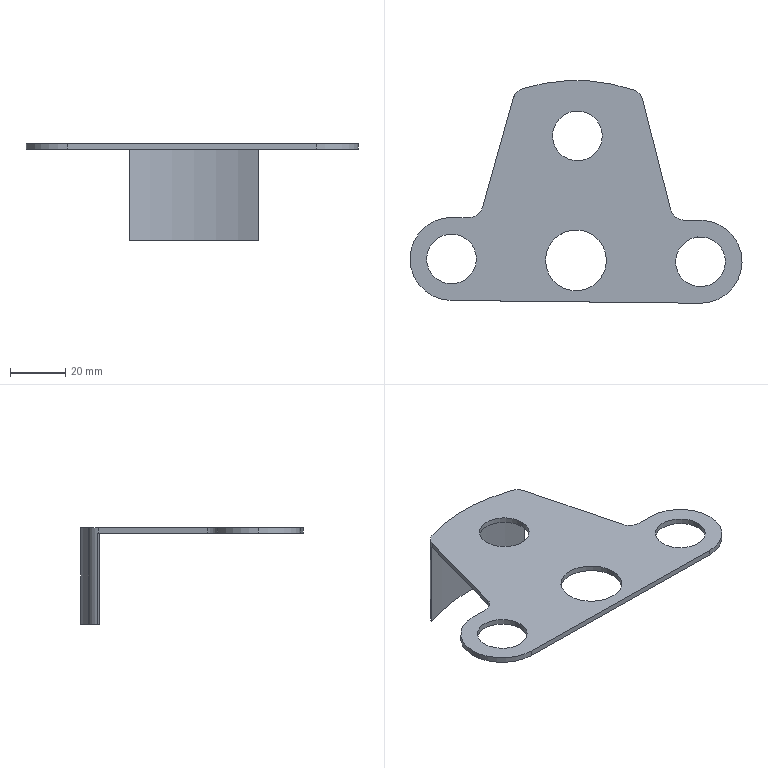Component | SolidWorks | JF21-80.2-34-1-SOLID1-1 | 1 solid | 26 faces | box 119.99 x 80.51 x 35 mm | volume 13117 mm3 | cylinder 18 | plane 8 | commonest cylinder face diameters 18 x6 30 x4 10 x4 22 x2 130 x1 126 x1
STEP:
#1=COLOUR_RGB('',0.7922,0.8196,0.9333);
#2=FILL_AREA_STYLE_COLOUR('',#1);
#3=FILL_AREA_STYLE('',(#2));
#4=SURFACE_STYLE_FILL_AREA(#3);
#5=SURFACE_SIDE_STYLE('',(#4));
#6=SURFACE_STYLE_USAGE(.BOTH.,#5);
#7=PRESENTATION_STYLE_ASSIGNMENT((#6));
#8=CARTESIAN_POINT('',(-1.765,0.6105,-11.063));
#9=VERTEX_POINT('',#8);
#10=CARTESIAN_POINT('',(-2.362,0.02663,-11.063));
#11=VERTEX_POINT('',#10);
#12=CARTESIAN_POINT('',(-1.772,0.01997,-11.063));
#13=DIRECTION('',(0.,0.,1.));
#14=DIRECTION('',(0.9999,-0.01127,0.));
#15=AXIS2_PLACEMENT_3D('',#12,#13,#14);
#16=CIRCLE('',#15,0.5906);
#17=EDGE_CURVE('',#9,#11,#16,.T.);
#18=ORIENTED_EDGE('',*,*,#17,.T.);
#19=CARTESIAN_POINT('',(-2.362,0.02663,-10.984));
#20=VERTEX_POINT('',#19);
#21=CARTESIAN_POINT('',(-2.362,0.02663,-11.063));
#22=DIRECTION('',(0.,0.,1.));
#23=VECTOR('',#22,39.37);
#24=LINE('',#21,#23);
#25=EDGE_CURVE('',#11,#20,#24,.T.);
#26=ORIENTED_EDGE('',*,*,#25,.T.);
#27=CARTESIAN_POINT('',(-1.765,0.6105,-10.984));
#28=VERTEX_POINT('',#27);
#29=CARTESIAN_POINT('',(-1.772,0.01997,-10.984));
#30=DIRECTION('',(0.,0.,1.));
#31=DIRECTION('',(0.9999,-0.01127,0.));
#32=AXIS2_PLACEMENT_3D('',#29,#30,#31);
#33=CIRCLE('',#32,0.5906);
#34=EDGE_CURVE('',#28,#20,#33,.T.);
#35=ORIENTED_EDGE('',*,*,#34,.F.);
#36=CARTESIAN_POINT('',(-1.765,0.6105,-11.063));
#37=DIRECTION('',(0.,0.,1.));
#38=VECTOR('',#37,39.37);
#39=LINE('',#36,#38);
#40=EDGE_CURVE('',#9,#28,#39,.T.);
#41=ORIENTED_EDGE('',*,*,#40,.F.);
#42=EDGE_LOOP('',(#18,#26,#35,#41));
#43=FACE_OUTER_BOUND('',#42,.T.);
#44=CARTESIAN_POINT('',(-1.772,0.01997,-11.063));
#45=DIRECTION('',(0.,0.,1.));
#46=DIRECTION('',(-0.9999,0.01127,0.));
#47=AXIS2_PLACEMENT_3D('',#44,#45,#46);
#48=CYLINDRICAL_SURFACE('',#47,0.5906);
#49=ADVANCED_FACE('',(#43),#48,.T.);
#50=CARTESIAN_POINT('',(-0.433,0.004883,-11.063));
#51=VERTEX_POINT('',#50);
#52=CARTESIAN_POINT('',(0.433,-0.004883,-11.063));
#53=VERTEX_POINT('',#52);
#54=CARTESIAN_POINT('',(0.,-0.,-11.063));
#55=DIRECTION('',(0.,0.,1.));
#56=DIRECTION('',(0.9999,-0.01127,0.));
#57=AXIS2_PLACEMENT_3D('',#54,#55,#56);
#58=CIRCLE('',#57,0.4331);
#59=EDGE_CURVE('',#51,#53,#58,.T.);
#60=ORIENTED_EDGE('',*,*,#59,.F.);
#61=CARTESIAN_POINT('',(-0.433,0.004883,-10.984));
#62=VERTEX_POINT('',#61);
#63=CARTESIAN_POINT('',(-0.433,0.004883,-11.063));
#64=DIRECTION('',(0.,0.,1.));
#65=VECTOR('',#64,39.37);
#66=LINE('',#63,#65);
#67=EDGE_CURVE('',#51,#62,#66,.T.);
#68=ORIENTED_EDGE('',*,*,#67,.T.);
#69=CARTESIAN_POINT('',(0.433,-0.004883,-10.984));
#70=VERTEX_POINT('',#69);
#71=CARTESIAN_POINT('',(0.,-0.,-10.984));
#72=DIRECTION('',(0.,0.,1.));
#73=DIRECTION('',(0.9999,-0.01127,0.));
#74=AXIS2_PLACEMENT_3D('',#71,#72,#73);
#75=CIRCLE('',#74,0.4331);
#76=EDGE_CURVE('',#62,#70,#75,.T.);
#77=ORIENTED_EDGE('',*,*,#76,.T.);
#78=CARTESIAN_POINT('',(0.433,-0.004883,-11.063));
#79=DIRECTION('',(0.,0.,1.));
#80=VECTOR('',#79,39.37);
#81=LINE('',#78,#80);
#82=EDGE_CURVE('',#53,#70,#81,.T.);
#83=ORIENTED_EDGE('',*,*,#82,.F.);
#84=EDGE_LOOP('',(#60,#68,#77,#83));
#85=FACE_OUTER_BOUND('',#84,.T.);
#86=CARTESIAN_POINT('',(0.,-0.,-11.063));
#87=DIRECTION('',(0.,0.,1.));
#88=DIRECTION('',(-0.9999,0.01127,0.));
#89=AXIS2_PLACEMENT_3D('',#86,#87,#88);
#90=CYLINDRICAL_SURFACE('',#89,0.4331);
#91=ADVANCED_FACE('',(#85),#90,.F.);
#92=CARTESIAN_POINT('',(1.417,-0.01598,-11.063));
#93=VERTEX_POINT('',#92);
#94=CARTESIAN_POINT('',(2.126,-0.02397,-11.063));
#95=VERTEX_POINT('',#94);
#96=CARTESIAN_POINT('',(1.772,-0.01997,-11.063));
#97=DIRECTION('',(0.,0.,1.));
#98=DIRECTION('',(0.9999,-0.01127,0.));
#99=AXIS2_PLACEMENT_3D('',#96,#97,#98);
#100=CIRCLE('',#99,0.3543);
#101=EDGE_CURVE('',#93,#95,#100,.T.);
#102=ORIENTED_EDGE('',*,*,#101,.F.);
#103=CARTESIAN_POINT('',(1.417,-0.01598,-10.984));
#104=VERTEX_POINT('',#103);
#105=CARTESIAN_POINT('',(1.417,-0.01598,-11.063));
#106=DIRECTION('',(0.,0.,1.));
#107=VECTOR('',#106,39.37);
#108=LINE('',#105,#107);
#109=EDGE_CURVE('',#93,#104,#108,.T.);
#110=ORIENTED_EDGE('',*,*,#109,.T.);
#111=CARTESIAN_POINT('',(2.126,-0.02397,-10.984));
#112=VERTEX_POINT('',#111);
#113=CARTESIAN_POINT('',(1.772,-0.01997,-10.984));
#114=DIRECTION('',(0.,0.,1.));
#115=DIRECTION('',(0.9999,-0.01127,0.));
#116=AXIS2_PLACEMENT_3D('',#113,#114,#115);
#117=CIRCLE('',#116,0.3543);
#118=EDGE_CURVE('',#104,#112,#117,.T.);
#119=ORIENTED_EDGE('',*,*,#118,.T.);
#120=CARTESIAN_POINT('',(2.126,-0.02397,-11.063));
#121=DIRECTION('',(0.,0.,1.));
#122=VECTOR('',#121,39.37);
#123=LINE('',#120,#122);
#124=EDGE_CURVE('',#95,#112,#123,.T.);
#125=ORIENTED_EDGE('',*,*,#124,.F.);
#126=EDGE_LOOP('',(#102,#110,#119,#125));
#127=FACE_OUTER_BOUND('',#126,.T.);
#128=CARTESIAN_POINT('',(1.772,-0.01997,-11.063));
#129=DIRECTION('',(0.,0.,1.));
#130=DIRECTION('',(-0.9999,0.01127,0.));
#131=AXIS2_PLACEMENT_3D('',#128,#129,#130);
#132=CYLINDRICAL_SURFACE('',#131,0.3543);
#133=ADVANCED_FACE('',(#127),#132,.F.);
#134=CARTESIAN_POINT('',(-2.126,0.02397,-11.063));
#135=VERTEX_POINT('',#134);
#136=CARTESIAN_POINT('',(-1.417,0.01598,-11.063));
#137=VERTEX_POINT('',#136);
#138=CARTESIAN_POINT('',(-1.772,0.01997,-11.063));
#139=DIRECTION('',(0.,0.,1.));
#140=DIRECTION('',(0.9999,-0.01127,0.));
#141=AXIS2_PLACEMENT_3D('',#138,#139,#140);
#142=CIRCLE('',#141,0.3543);
#143=EDGE_CURVE('',#135,#137,#142,.T.);
#144=ORIENTED_EDGE('',*,*,#143,.F.);
#145=CARTESIAN_POINT('',(-2.126,0.02397,-10.984));
#146=VERTEX_POINT('',#145);
#147=CARTESIAN_POINT('',(-2.126,0.02397,-11.063));
#148=DIRECTION('',(0.,0.,1.));
#149=VECTOR('',#148,39.37);
#150=LINE('',#147,#149);
#151=EDGE_CURVE('',#135,#146,#150,.T.);
#152=ORIENTED_EDGE('',*,*,#151,.T.);
#153=CARTESIAN_POINT('',(-1.417,0.01598,-10.984));
#154=VERTEX_POINT('',#153);
#155=CARTESIAN_POINT('',(-1.772,0.01997,-10.984));
#156=DIRECTION('',(0.,0.,1.));
#157=DIRECTION('',(0.9999,-0.01127,0.));
#158=AXIS2_PLACEMENT_3D('',#155,#156,#157);
#159=CIRCLE('',#158,0.3543);
#160=EDGE_CURVE('',#146,#154,#159,.T.);
#161=ORIENTED_EDGE('',*,*,#160,.T.);
#162=CARTESIAN_POINT('',(-1.417,0.01598,-11.063));
#163=DIRECTION('',(0.,0.,1.));
#164=VECTOR('',#163,39.37);
#165=LINE('',#162,#164);
#166=EDGE_CURVE('',#137,#154,#165,.T.);
#167=ORIENTED_EDGE('',*,*,#166,.F.);
#168=EDGE_LOOP('',(#144,#152,#161,#167));
#169=FACE_OUTER_BOUND('',#168,.T.);
#170=CARTESIAN_POINT('',(-1.772,0.01997,-11.063));
#171=DIRECTION('',(0.,0.,1.));
#172=DIRECTION('',(-0.9999,0.01127,0.));
#173=AXIS2_PLACEMENT_3D('',#170,#171,#172);
#174=CYLINDRICAL_SURFACE('',#173,0.3543);
#175=ADVANCED_FACE('',(#169),#174,.F.);
#176=CARTESIAN_POINT('',(-0.3343,1.776,-11.063));
#177=VERTEX_POINT('',#176);
#178=CARTESIAN_POINT('',(0.3743,1.768,-11.063));
#179=VERTEX_POINT('',#178);
#180=CARTESIAN_POINT('',(0.01997,1.772,-11.063));
#181=DIRECTION('',(0.,0.,1.));
#182=DIRECTION('',(0.9999,-0.01127,0.));
#183=AXIS2_PLACEMENT_3D('',#180,#181,#182);
#184=CIRCLE('',#183,0.3543);
#185=EDGE_CURVE('',#177,#179,#184,.T.);
#186=ORIENTED_EDGE('',*,*,#185,.F.);
#187=CARTESIAN_POINT('',(-0.3343,1.776,-10.984));
#188=VERTEX_POINT('',#187);
#189=CARTESIAN_POINT('',(-0.3343,1.776,-11.063));
#190=DIRECTION('',(0.,0.,1.));
#191=VECTOR('',#190,39.37);
#192=LINE('',#189,#191);
#193=EDGE_CURVE('',#177,#188,#192,.T.);
#194=ORIENTED_EDGE('',*,*,#193,.T.);
#195=CARTESIAN_POINT('',(0.3743,1.768,-10.984));
#196=VERTEX_POINT('',#195);
#197=CARTESIAN_POINT('',(0.01997,1.772,-10.984));
#198=DIRECTION('',(0.,0.,1.));
#199=DIRECTION('',(0.9999,-0.01127,0.));
#200=AXIS2_PLACEMENT_3D('',#197,#198,#199);
#201=CIRCLE('',#200,0.3543);
#202=EDGE_CURVE('',#188,#196,#201,.T.);
#203=ORIENTED_EDGE('',*,*,#202,.T.);
#204=CARTESIAN_POINT('',(0.3743,1.768,-11.063));
#205=DIRECTION('',(0.,0.,1.));
#206=VECTOR('',#205,39.37);
#207=LINE('',#204,#206);
#208=EDGE_CURVE('',#179,#196,#207,.T.);
#209=ORIENTED_EDGE('',*,*,#208,.F.);
#210=EDGE_LOOP('',(#186,#194,#203,#209));
#211=FACE_OUTER_BOUND('',#210,.T.);
#212=CARTESIAN_POINT('',(0.01997,1.772,-11.063));
#213=DIRECTION('',(0.,0.,1.));
#214=DIRECTION('',(-0.9999,0.01127,0.));
#215=AXIS2_PLACEMENT_3D('',#212,#213,#214);
#216=CYLINDRICAL_SURFACE('',#215,0.3543);
#217=ADVANCED_FACE('',(#211),#216,.F.);
#218=CARTESIAN_POINT('',(1.765,-0.6105,-11.063));
#219=VERTEX_POINT('',#218);
#220=CARTESIAN_POINT('',(2.362,-0.02663,-11.063));
#221=VERTEX_POINT('',#220);
#222=CARTESIAN_POINT('',(1.772,-0.01997,-11.063));
#223=DIRECTION('',(0.,0.,1.));
#224=DIRECTION('',(-0.9999,0.01127,0.));
#225=AXIS2_PLACEMENT_3D('',#222,#223,#224);
#226=CIRCLE('',#225,0.5906);
#227=EDGE_CURVE('',#219,#221,#226,.T.);
#228=ORIENTED_EDGE('',*,*,#227,.T.);
#229=CARTESIAN_POINT('',(2.362,-0.02663,-10.984));
#230=VERTEX_POINT('',#229);
#231=CARTESIAN_POINT('',(2.362,-0.02663,-11.063));
#232=DIRECTION('',(0.,0.,1.));
#233=VECTOR('',#232,39.37);
#234=LINE('',#231,#233);
#235=EDGE_CURVE('',#221,#230,#234,.T.);
#236=ORIENTED_EDGE('',*,*,#235,.T.);
#237=CARTESIAN_POINT('',(1.765,-0.6105,-10.984));
#238=VERTEX_POINT('',#237);
#239=CARTESIAN_POINT('',(1.772,-0.01997,-10.984));
#240=DIRECTION('',(0.,0.,1.));
#241=DIRECTION('',(-0.9999,0.01127,0.));
#242=AXIS2_PLACEMENT_3D('',#239,#240,#241);
#243=CIRCLE('',#242,0.5906);
#244=EDGE_CURVE('',#238,#230,#243,.T.);
#245=ORIENTED_EDGE('',*,*,#244,.F.);
#246=CARTESIAN_POINT('',(1.765,-0.6105,-11.063));
#247=DIRECTION('',(0.,0.,1.));
#248=VECTOR('',#247,39.37);
#249=LINE('',#246,#248);
#250=EDGE_CURVE('',#219,#238,#249,.T.);
#251=ORIENTED_EDGE('',*,*,#250,.F.);
#252=EDGE_LOOP('',(#228,#236,#245,#251));
#253=FACE_OUTER_BOUND('',#252,.T.);
#254=CARTESIAN_POINT('',(1.772,-0.01997,-11.063));
#255=DIRECTION('',(0.,0.,1.));
#256=DIRECTION('',(-0.9999,0.01127,0.));
#257=AXIS2_PLACEMENT_3D('',#254,#255,#256);
#258=CYLINDRICAL_SURFACE('',#257,0.5906);
#259=ADVANCED_FACE('',(#253),#258,.T.);
#260=ORIENTED_EDGE('',*,*,#235,.F.);
#261=CARTESIAN_POINT('',(1.778,0.5705,-11.063));
#262=VERTEX_POINT('',#261);
#263=CARTESIAN_POINT('',(1.772,-0.01997,-11.063));
#264=DIRECTION('',(0.,0.,1.));
#265=DIRECTION('',(-0.9999,0.01127,0.));
#266=AXIS2_PLACEMENT_3D('',#263,#264,#265);
#267=CIRCLE('',#266,0.5906);
#268=EDGE_CURVE('',#221,#262,#267,.T.);
#269=ORIENTED_EDGE('',*,*,#268,.T.);
#270=CARTESIAN_POINT('',(1.778,0.5705,-10.984));
#271=VERTEX_POINT('',#270);
#272=CARTESIAN_POINT('',(1.778,0.5705,-11.063));
#273=DIRECTION('',(0.,0.,1.));
#274=VECTOR('',#273,39.37);
#275=LINE('',#272,#274);
#276=EDGE_CURVE('',#262,#271,#275,.T.);
#277=ORIENTED_EDGE('',*,*,#276,.T.);
#278=CARTESIAN_POINT('',(1.772,-0.01997,-10.984));
#279=DIRECTION('',(0.,0.,1.));
#280=DIRECTION('',(-0.9999,0.01127,0.));
#281=AXIS2_PLACEMENT_3D('',#278,#279,#280);
#282=CIRCLE('',#281,0.5906);
#283=EDGE_CURVE('',#230,#271,#282,.T.);
#284=ORIENTED_EDGE('',*,*,#283,.F.);
#285=EDGE_LOOP('',(#260,#269,#277,#284));
#286=FACE_OUTER_BOUND('',#285,.T.);
#287=CARTESIAN_POINT('',(1.772,-0.01997,-11.063));
#288=DIRECTION('',(0.,0.,1.));
#289=DIRECTION('',(-0.9999,0.01127,0.));
#290=AXIS2_PLACEMENT_3D('',#287,#288,#289);
#291=CYLINDRICAL_SURFACE('',#290,0.5906);
#292=ADVANCED_FACE('',(#286),#291,.T.);
#293=CARTESIAN_POINT('',(-1.778,-0.5705,-10.984));
#294=VERTEX_POINT('',#293);
#295=CARTESIAN_POINT('',(-1.778,-0.5705,-10.984));
#296=DIRECTION('',(0.9999,-0.01127,0.));
#297=VECTOR('',#296,39.37);
#298=LINE('',#295,#297);
#299=EDGE_CURVE('',#294,#238,#298,.T.);
#300=ORIENTED_EDGE('',*,*,#299,.F.);
#301=CARTESIAN_POINT('',(-1.778,-0.5705,-11.063));
#302=VERTEX_POINT('',#301);
#303=CARTESIAN_POINT('',(-1.778,-0.5705,-11.063));
#304=DIRECTION('',(0.,0.,1.));
#305=VECTOR('',#304,39.37);
#306=LINE('',#303,#305);
#307=EDGE_CURVE('',#302,#294,#306,.T.);
#308=ORIENTED_EDGE('',*,*,#307,.F.);
#309=CARTESIAN_POINT('',(-1.778,-0.5705,-11.063));
#310=DIRECTION('',(0.9999,-0.01127,0.));
#311=VECTOR('',#310,39.37);
#312=LINE('',#309,#311);
#313=EDGE_CURVE('',#302,#219,#312,.T.);
#314=ORIENTED_EDGE('',*,*,#313,.T.);
#315=ORIENTED_EDGE('',*,*,#250,.T.);
#316=EDGE_LOOP('',(#300,#308,#314,#315));
#317=FACE_OUTER_BOUND('',#316,.T.);
#318=CARTESIAN_POINT('',(-1.778,-0.5705,-11.063));
#319=DIRECTION('',(-0.01127,-0.9999,0.));
#320=DIRECTION('',(0.,0.,1.));
#321=AXIS2_PLACEMENT_3D('',#318,#319,#320);
#322=PLANE('',#321);
#323=ADVANCED_FACE('',(#317),#322,.T.);
#324=ORIENTED_EDGE('',*,*,#25,.F.);
#325=CARTESIAN_POINT('',(-1.772,0.01997,-11.063));
#326=DIRECTION('',(0.,0.,1.));
#327=DIRECTION('',(0.9999,-0.01127,0.));
#328=AXIS2_PLACEMENT_3D('',#325,#326,#327);
#329=CIRCLE('',#328,0.5906);
#330=EDGE_CURVE('',#11,#302,#329,.T.);
#331=ORIENTED_EDGE('',*,*,#330,.T.);
#332=ORIENTED_EDGE('',*,*,#307,.T.);
#333=CARTESIAN_POINT('',(-1.772,0.01997,-10.984));
#334=DIRECTION('',(0.,0.,1.));
#335=DIRECTION('',(0.9999,-0.01127,0.));
#336=AXIS2_PLACEMENT_3D('',#333,#334,#335);
#337=CIRCLE('',#336,0.5906);
#338=EDGE_CURVE('',#20,#294,#337,.T.);
#339=ORIENTED_EDGE('',*,*,#338,.F.);
#340=EDGE_LOOP('',(#324,#331,#332,#339));
#341=FACE_OUTER_BOUND('',#340,.T.);
#342=CARTESIAN_POINT('',(-1.772,0.01997,-11.063));
#343=DIRECTION('',(0.,0.,1.));
#344=DIRECTION('',(-0.9999,0.01127,0.));
#345=AXIS2_PLACEMENT_3D('',#342,#343,#344);
#346=CYLINDRICAL_SURFACE('',#345,0.5906);
#347=ADVANCED_FACE('',(#341),#346,.T.);
#348=CARTESIAN_POINT('',(-1.522,0.6078,-10.984));
#349=VERTEX_POINT('',#348);
#350=CARTESIAN_POINT('',(-1.765,0.6105,-10.984));
#351=DIRECTION('',(-0.9999,0.01127,0.));
#352=VECTOR('',#351,39.37);
#353=LINE('',#350,#352);
#354=EDGE_CURVE('',#349,#28,#353,.T.);
#355=ORIENTED_EDGE('',*,*,#354,.F.);
#356=CARTESIAN_POINT('',(-1.522,0.6078,-11.063));
#357=VERTEX_POINT('',#356);
#358=CARTESIAN_POINT('',(-1.522,0.6078,-11.063));
#359=DIRECTION('',(0.,0.,1.));
#360=VECTOR('',#359,39.37);
#361=LINE('',#358,#360);
#362=EDGE_CURVE('',#357,#349,#361,.T.);
#363=ORIENTED_EDGE('',*,*,#362,.F.);
#364=CARTESIAN_POINT('',(-1.765,0.6105,-11.063));
#365=DIRECTION('',(-0.9999,0.01127,0.));
#366=VECTOR('',#365,39.37);
#367=LINE('',#364,#366);
#368=EDGE_CURVE('',#357,#9,#367,.T.);
#369=ORIENTED_EDGE('',*,*,#368,.T.);
#370=ORIENTED_EDGE('',*,*,#40,.T.);
#371=EDGE_LOOP('',(#355,#363,#369,#370));
#372=FACE_OUTER_BOUND('',#371,.T.);
#373=CARTESIAN_POINT('',(-1.765,0.6105,-11.063));
#374=DIRECTION('',(0.01127,0.9999,0.));
#375=DIRECTION('',(0.9999,-0.01127,0.));
#376=AXIS2_PLACEMENT_3D('',#373,#374,#375);
#377=PLANE('',#376);
#378=ADVANCED_FACE('',(#372),#377,.T.);
#379=CARTESIAN_POINT('',(-1.33,0.7515,-10.984));
#380=VERTEX_POINT('',#379);
#381=CARTESIAN_POINT('',(-1.52,0.8046,-10.984));
#382=DIRECTION('',(0.,0.,-1.));
#383=DIRECTION('',(0.9999,-0.01127,0.));
#384=AXIS2_PLACEMENT_3D('',#381,#382,#383);
#385=CIRCLE('',#384,0.1969);
#386=EDGE_CURVE('',#380,#349,#385,.T.);
#387=ORIENTED_EDGE('',*,*,#386,.F.);
#388=CARTESIAN_POINT('',(-1.33,0.7515,-11.063));
#389=VERTEX_POINT('',#388);
#390=CARTESIAN_POINT('',(-1.33,0.7515,-11.063));
#391=DIRECTION('',(0.,0.,1.));
#392=VECTOR('',#391,39.37);
#393=LINE('',#390,#392);
#394=EDGE_CURVE('',#389,#380,#393,.T.);
#395=ORIENTED_EDGE('',*,*,#394,.F.);
#396=CARTESIAN_POINT('',(-1.52,0.8046,-11.063));
#397=DIRECTION('',(0.,0.,-1.));
#398=DIRECTION('',(0.9999,-0.01127,0.));
#399=AXIS2_PLACEMENT_3D('',#396,#397,#398);
#400=CIRCLE('',#399,0.1969);
#401=EDGE_CURVE('',#389,#357,#400,.T.);
#402=ORIENTED_EDGE('',*,*,#401,.T.);
#403=ORIENTED_EDGE('',*,*,#362,.T.);
#404=EDGE_LOOP('',(#387,#395,#402,#403));
#405=FACE_OUTER_BOUND('',#404,.T.);
#406=CARTESIAN_POINT('',(-1.52,0.8046,-11.063));
#407=DIRECTION('',(0.,0.,1.));
#408=DIRECTION('',(-0.9999,0.01127,0.));
#409=AXIS2_PLACEMENT_3D('',#406,#407,#408);
#410=CYLINDRICAL_SURFACE('',#409,0.1969);
#411=ADVANCED_FACE('',(#405),#410,.F.);
#412=CARTESIAN_POINT('',(-0.8947,2.308,-10.984));
#413=VERTEX_POINT('',#412);
#414=CARTESIAN_POINT('',(-1.33,0.7515,-10.984));
#415=DIRECTION('',(-0.2697,-0.9629,0.));
#416=VECTOR('',#415,39.37);
#417=LINE('',#414,#416);
#418=EDGE_CURVE('',#413,#380,#417,.T.);
#419=ORIENTED_EDGE('',*,*,#418,.F.);
#420=CARTESIAN_POINT('',(-0.8947,2.308,-11.063));
#421=VERTEX_POINT('',#420);
#422=CARTESIAN_POINT('',(-0.8947,2.308,-11.063));
#423=DIRECTION('',(0.,0.,1.));
#424=VECTOR('',#423,39.37);
#425=LINE('',#422,#424);
#426=EDGE_CURVE('',#421,#413,#425,.T.);
#427=ORIENTED_EDGE('',*,*,#426,.F.);
#428=CARTESIAN_POINT('',(-1.33,0.7515,-11.063));
#429=DIRECTION('',(-0.2697,-0.9629,0.));
#430=VECTOR('',#429,39.37);
#431=LINE('',#428,#430);
#432=EDGE_CURVE('',#421,#389,#431,.T.);
#433=ORIENTED_EDGE('',*,*,#432,.T.);
#434=ORIENTED_EDGE('',*,*,#394,.T.);
#435=EDGE_LOOP('',(#419,#427,#433,#434));
#436=FACE_OUTER_BOUND('',#435,.T.);
#437=CARTESIAN_POINT('',(-1.33,0.7515,-11.063));
#438=DIRECTION('',(-0.9629,0.2697,0.));
#439=DIRECTION('',(0.2697,0.9629,0.));
#440=AXIS2_PLACEMENT_3D('',#437,#438,#439);
#441=PLANE('',#440);
#442=ADVANCED_FACE('',(#436),#441,.T.);
#443=CARTESIAN_POINT('',(-0.7639,2.442,-10.984));
#444=VERTEX_POINT('',#443);
#445=CARTESIAN_POINT('',(-0.7051,2.255,-10.984));
#446=DIRECTION('',(0.,0.,1.));
#447=DIRECTION('',(-0.9999,0.01127,0.));
#448=AXIS2_PLACEMENT_3D('',#445,#446,#447);
#449=CIRCLE('',#448,0.1969);
#450=EDGE_CURVE('',#444,#413,#449,.T.);
#451=ORIENTED_EDGE('',*,*,#450,.F.);
#452=CARTESIAN_POINT('',(-0.7639,2.442,-12.362));
#453=VERTEX_POINT('',#452);
#454=CARTESIAN_POINT('',(-0.7639,2.442,-11.063));
#455=DIRECTION('',(0.,0.,1.));
#456=VECTOR('',#455,39.37);
#457=LINE('',#454,#456);
#458=EDGE_CURVE('',#453,#444,#457,.T.);
#459=ORIENTED_EDGE('',*,*,#458,.F.);
#460=CARTESIAN_POINT('',(-0.8927,2.314,-12.362));
#461=VERTEX_POINT('',#460);
#462=CARTESIAN_POINT('',(-0.7051,2.255,-12.362));
#463=DIRECTION('',(0.,0.,-1.));
#464=DIRECTION('',(-0.9999,0.01127,0.));
#465=AXIS2_PLACEMENT_3D('',#462,#463,#464);
#466=CIRCLE('',#465,0.1969);
#467=EDGE_CURVE('',#461,#453,#466,.T.);
#468=ORIENTED_EDGE('',*,*,#467,.F.);
#469=CARTESIAN_POINT('',(-0.8927,2.314,-11.063));
#470=VERTEX_POINT('',#469);
#471=CARTESIAN_POINT('',(-0.8927,2.314,-12.362));
#472=DIRECTION('',(0.,0.,1.));
#473=VECTOR('',#472,39.37);
#474=LINE('',#471,#473);
#475=EDGE_CURVE('',#461,#470,#474,.T.);
#476=ORIENTED_EDGE('',*,*,#475,.T.);
#477=CARTESIAN_POINT('',(-0.7051,2.255,-11.063));
#478=DIRECTION('',(0.,0.,1.));
#479=DIRECTION('',(-0.9999,0.01127,0.));
#480=AXIS2_PLACEMENT_3D('',#477,#478,#479);
#481=CIRCLE('',#480,0.1969);
#482=EDGE_CURVE('',#470,#421,#481,.T.);
#483=ORIENTED_EDGE('',*,*,#482,.T.);
#484=ORIENTED_EDGE('',*,*,#426,.T.);
#485=EDGE_LOOP('',(#451,#459,#468,#476,#483,#484));
#486=FACE_OUTER_BOUND('',#485,.T.);
#487=CARTESIAN_POINT('',(-0.7051,2.255,-11.063));
#488=DIRECTION('',(0.,0.,1.));
#489=DIRECTION('',(-0.9999,0.01127,0.));
#490=AXIS2_PLACEMENT_3D('',#487,#488,#489);
#491=CYLINDRICAL_SURFACE('',#490,0.1969);
#492=ADVANCED_FACE('',(#486),#491,.T.);
#493=CARTESIAN_POINT('',(0.8187,2.425,-10.984));
#494=VERTEX_POINT('',#493);
#495=CARTESIAN_POINT('',(0.,-0.,-10.984));
#496=DIRECTION('',(0.,0.,1.));
#497=DIRECTION('',(-0.9999,0.01127,0.));
#498=AXIS2_PLACEMENT_3D('',#495,#496,#497);
#499=CIRCLE('',#498,2.559);
#500=EDGE_CURVE('',#494,#444,#499,.T.);
#501=ORIENTED_EDGE('',*,*,#500,.F.);
#502=CARTESIAN_POINT('',(0.8187,2.425,-12.362));
#503=VERTEX_POINT('',#502);
#504=CARTESIAN_POINT('',(0.8187,2.425,-11.063));
#505=DIRECTION('',(0.,0.,1.));
#506=VECTOR('',#505,39.37);
#507=LINE('',#504,#506);
#508=EDGE_CURVE('',#503,#494,#507,.T.);
#509=ORIENTED_EDGE('',*,*,#508,.F.);
#510=CARTESIAN_POINT('',(0.,-0.,-12.362));
#511=DIRECTION('',(0.,0.,-1.));
#512=DIRECTION('',(-0.9999,0.01127,0.));
#513=AXIS2_PLACEMENT_3D('',#510,#511,#512);
#514=CIRCLE('',#513,2.559);
#515=EDGE_CURVE('',#453,#503,#514,.T.);
#516=ORIENTED_EDGE('',*,*,#515,.F.);
#517=ORIENTED_EDGE('',*,*,#458,.T.);
#518=EDGE_LOOP('',(#501,#509,#516,#517));
#519=FACE_OUTER_BOUND('',#518,.T.);
#520=CARTESIAN_POINT('',(0.,-0.,-11.063));
#521=DIRECTION('',(0.,0.,1.));
#522=DIRECTION('',(-0.9999,0.01127,0.));
#523=AXIS2_PLACEMENT_3D('',#520,#521,#522);
#524=CYLINDRICAL_SURFACE('',#523,2.559);
#525=ADVANCED_FACE('',(#519),#524,.T.);
#526=CARTESIAN_POINT('',(0.9465,2.287,-10.984));
#527=VERTEX_POINT('',#526);
#528=CARTESIAN_POINT('',(0.7557,2.238,-10.984));
#529=DIRECTION('',(0.,0.,1.));
#530=DIRECTION('',(0.9999,-0.01127,0.));
#531=AXIS2_PLACEMENT_3D('',#528,#529,#530);
#532=CIRCLE('',#531,0.1969);
#533=EDGE_CURVE('',#527,#494,#532,.T.);
#534=ORIENTED_EDGE('',*,*,#533,.F.);
#535=CARTESIAN_POINT('',(0.9465,2.287,-11.063));
#536=VERTEX_POINT('',#535);
#537=CARTESIAN_POINT('',(0.9465,2.287,-11.063));
#538=DIRECTION('',(0.,0.,1.));
#539=VECTOR('',#538,39.37);
#540=LINE('',#537,#539);
#541=EDGE_CURVE('',#536,#527,#540,.T.);
#542=ORIENTED_EDGE('',*,*,#541,.F.);
#543=CARTESIAN_POINT('',(0.9447,2.293,-11.063));
#544=VERTEX_POINT('',#543);
#545=CARTESIAN_POINT('',(0.7557,2.238,-11.063));
#546=DIRECTION('',(0.,0.,1.));
#547=DIRECTION('',(0.9999,-0.01127,0.));
#548=AXIS2_PLACEMENT_3D('',#545,#546,#547);
#549=CIRCLE('',#548,0.1969);
#550=EDGE_CURVE('',#536,#544,#549,.T.);
#551=ORIENTED_EDGE('',*,*,#550,.T.);
#552=CARTESIAN_POINT('',(0.9447,2.293,-12.362));
#553=VERTEX_POINT('',#552);
#554=CARTESIAN_POINT('',(0.9447,2.293,-12.362));
#555=DIRECTION('',(0.,0.,1.));
#556=VECTOR('',#555,39.37);
#557=LINE('',#554,#556);
#558=EDGE_CURVE('',#553,#544,#557,.T.);
#559=ORIENTED_EDGE('',*,*,#558,.F.);
#560=CARTESIAN_POINT('',(0.7557,2.238,-12.362));
#561=DIRECTION('',(0.,0.,-1.));
#562=DIRECTION('',(-0.9999,0.01127,0.));
#563=AXIS2_PLACEMENT_3D('',#560,#561,#562);
#564=CIRCLE('',#563,0.1969);
#565=EDGE_CURVE('',#503,#553,#564,.T.);
#566=ORIENTED_EDGE('',*,*,#565,.F.);
#567=ORIENTED_EDGE('',*,*,#508,.T.);
#568=EDGE_LOOP('',(#534,#542,#551,#559,#566,#567));
#569=FACE_OUTER_BOUND('',#568,.T.);
#570=CARTESIAN_POINT('',(0.7557,2.238,-11.063));
#571=DIRECTION('',(0.,0.,1.));
#572=DIRECTION('',(-0.9999,0.01127,0.));
#573=AXIS2_PLACEMENT_3D('',#570,#571,#572);
#574=CYLINDRICAL_SURFACE('',#573,0.1969);
#575=ADVANCED_FACE('',(#569),#574,.T.);
#576=CARTESIAN_POINT('',(1.347,0.7213,-10.984));
#577=VERTEX_POINT('',#576);
#578=CARTESIAN_POINT('',(1.347,0.7213,-10.984));
#579=DIRECTION('',(-0.2479,0.9688,0.));
#580=VECTOR('',#579,39.37);
#581=LINE('',#578,#580);
#582=EDGE_CURVE('',#577,#527,#581,.T.);
#583=ORIENTED_EDGE('',*,*,#582,.F.);
#584=CARTESIAN_POINT('',(1.347,0.7213,-11.063));
#585=VERTEX_POINT('',#584);
#586=CARTESIAN_POINT('',(1.347,0.7213,-11.063));
#587=DIRECTION('',(0.,0.,1.));
#588=VECTOR('',#587,39.37);
#589=LINE('',#586,#588);
#590=EDGE_CURVE('',#585,#577,#589,.T.);
#591=ORIENTED_EDGE('',*,*,#590,.F.);
#592=CARTESIAN_POINT('',(1.347,0.7213,-11.063));
#593=DIRECTION('',(-0.2479,0.9688,0.));
#594=VECTOR('',#593,39.37);
#595=LINE('',#592,#594);
#596=EDGE_CURVE('',#585,#536,#595,.T.);
#597=ORIENTED_EDGE('',*,*,#596,.T.);
#598=ORIENTED_EDGE('',*,*,#541,.T.);
#599=EDGE_LOOP('',(#583,#591,#597,#598));
#600=FACE_OUTER_BOUND('',#599,.T.);
#601=CARTESIAN_POINT('',(1.347,0.7213,-11.063));
#602=DIRECTION('',(0.9688,0.2479,0.));
#603=DIRECTION('',(0.2479,-0.9688,0.));
#604=AXIS2_PLACEMENT_3D('',#601,#602,#603);
#605=PLANE('',#604);
#606=ADVANCED_FACE('',(#600),#605,.T.);
#607=CARTESIAN_POINT('',(1.536,0.5733,-10.984));
#608=VERTEX_POINT('',#607);
#609=CARTESIAN_POINT('',(1.538,0.7701,-10.984));
#610=DIRECTION('',(0.,0.,-1.));
#611=DIRECTION('',(-0.9999,0.01127,0.));
#612=AXIS2_PLACEMENT_3D('',#609,#610,#611);
#613=CIRCLE('',#612,0.1969);
#614=EDGE_CURVE('',#608,#577,#613,.T.);
#615=ORIENTED_EDGE('',*,*,#614,.F.);
#616=CARTESIAN_POINT('',(1.536,0.5733,-11.063));
#617=VERTEX_POINT('',#616);
#618=CARTESIAN_POINT('',(1.536,0.5733,-11.063));
#619=DIRECTION('',(0.,0.,1.));
#620=VECTOR('',#619,39.37);
#621=LINE('',#618,#620);
#622=EDGE_CURVE('',#617,#608,#621,.T.);
#623=ORIENTED_EDGE('',*,*,#622,.F.);
#624=CARTESIAN_POINT('',(1.538,0.7701,-11.063));
#625=DIRECTION('',(0.,0.,-1.));
#626=DIRECTION('',(-0.9999,0.01127,0.));
#627=AXIS2_PLACEMENT_3D('',#624,#625,#626);
#628=CIRCLE('',#627,0.1969);
#629=EDGE_CURVE('',#617,#585,#628,.T.);
#630=ORIENTED_EDGE('',*,*,#629,.T.);
#631=ORIENTED_EDGE('',*,*,#590,.T.);
#632=EDGE_LOOP('',(#615,#623,#630,#631));
#633=FACE_OUTER_BOUND('',#632,.T.);
#634=CARTESIAN_POINT('',(1.538,0.7701,-11.063));
#635=DIRECTION('',(0.,0.,1.));
#636=DIRECTION('',(-0.9999,0.01127,0.));
#637=AXIS2_PLACEMENT_3D('',#634,#635,#636);
#638=CYLINDRICAL_SURFACE('',#637,0.1969);
#639=ADVANCED_FACE('',(#633),#638,.F.);
#640=CARTESIAN_POINT('',(1.778,0.5705,-10.984));
#641=DIRECTION('',(-0.9999,0.01127,0.));
#642=VECTOR('',#641,39.37);
#643=LINE('',#640,#642);
#644=EDGE_CURVE('',#271,#608,#643,.T.);
#645=ORIENTED_EDGE('',*,*,#644,.F.);
#646=ORIENTED_EDGE('',*,*,#276,.F.);
#647=CARTESIAN_POINT('',(1.778,0.5705,-11.063));
#648=DIRECTION('',(-0.9999,0.01127,0.));
#649=VECTOR('',#648,39.37);
#650=LINE('',#647,#649);
#651=EDGE_CURVE('',#262,#617,#650,.T.);
#652=ORIENTED_EDGE('',*,*,#651,.T.);
#653=ORIENTED_EDGE('',*,*,#622,.T.);
#654=EDGE_LOOP('',(#645,#646,#652,#653));
#655=FACE_OUTER_BOUND('',#654,.T.);
#656=CARTESIAN_POINT('',(1.778,0.5705,-11.063));
#657=DIRECTION('',(0.01127,0.9999,0.));
#658=DIRECTION('',(0.,0.,-1.));
#659=AXIS2_PLACEMENT_3D('',#656,#657,#658);
#660=PLANE('',#659);
#661=ADVANCED_FACE('',(#655),#660,.T.);
#662=CARTESIAN_POINT('',(0.,-0.,-11.063));
#663=DIRECTION('',(0.,0.,1.));
#664=DIRECTION('',(0.9999,-0.01127,0.));
#665=AXIS2_PLACEMENT_3D('',#662,#663,#664);
#666=CIRCLE('',#665,2.48);
#667=EDGE_CURVE('',#544,#470,#666,.T.);
#668=ORIENTED_EDGE('',*,*,#667,.F.);
#669=ORIENTED_EDGE('',*,*,#550,.F.);
#670=ORIENTED_EDGE('',*,*,#596,.F.);
#671=ORIENTED_EDGE('',*,*,#629,.F.);
#672=ORIENTED_EDGE('',*,*,#651,.F.);
#673=ORIENTED_EDGE('',*,*,#268,.F.);
#674=ORIENTED_EDGE('',*,*,#227,.F.);
#675=ORIENTED_EDGE('',*,*,#313,.F.);
#676=ORIENTED_EDGE('',*,*,#330,.F.);
#677=ORIENTED_EDGE('',*,*,#17,.F.);
#678=ORIENTED_EDGE('',*,*,#368,.F.);
#679=ORIENTED_EDGE('',*,*,#401,.F.);
#680=ORIENTED_EDGE('',*,*,#432,.F.);
#681=ORIENTED_EDGE('',*,*,#482,.F.);
#682=EDGE_LOOP('',(#668,#669,#670,#671,#672,#673,#674,#675,#676,#677,#678,#679,#680,#681));
#683=FACE_OUTER_BOUND('',#682,.T.);
#684=CARTESIAN_POINT('',(0.,-0.,-11.063));
#685=DIRECTION('',(0.,0.,1.));
#686=DIRECTION('',(0.9999,-0.01127,0.));
#687=AXIS2_PLACEMENT_3D('',#684,#685,#686);
#688=CIRCLE('',#687,0.4331);
#689=EDGE_CURVE('',#53,#51,#688,.T.);
#690=ORIENTED_EDGE('',*,*,#689,.T.);
#691=ORIENTED_EDGE('',*,*,#59,.T.);
#692=EDGE_LOOP('',(#690,#691));
#693=FACE_BOUND('',#692,.T.);
#694=CARTESIAN_POINT('',(1.772,-0.01997,-11.063));
#695=DIRECTION('',(0.,0.,1.));
#696=DIRECTION('',(0.9999,-0.01127,0.));
#697=AXIS2_PLACEMENT_3D('',#694,#695,#696);
#698=CIRCLE('',#697,0.3543);
#699=EDGE_CURVE('',#95,#93,#698,.T.);
#700=ORIENTED_EDGE('',*,*,#699,.T.);
#701=ORIENTED_EDGE('',*,*,#101,.T.);
#702=EDGE_LOOP('',(#700,#701));
#703=FACE_BOUND('',#702,.T.);
#704=CARTESIAN_POINT('',(-1.772,0.01997,-11.063));
#705=DIRECTION('',(0.,0.,1.));
#706=DIRECTION('',(0.9999,-0.01127,0.));
#707=AXIS2_PLACEMENT_3D('',#704,#705,#706);
#708=CIRCLE('',#707,0.3543);
#709=EDGE_CURVE('',#137,#135,#708,.T.);
#710=ORIENTED_EDGE('',*,*,#709,.T.);
#711=ORIENTED_EDGE('',*,*,#143,.T.);
#712=EDGE_LOOP('',(#710,#711));
#713=FACE_BOUND('',#712,.T.);
#714=CARTESIAN_POINT('',(0.01997,1.772,-11.063));
#715=DIRECTION('',(0.,0.,1.));
#716=DIRECTION('',(0.9999,-0.01127,0.));
#717=AXIS2_PLACEMENT_3D('',#714,#715,#716);
#718=CIRCLE('',#717,0.3543);
#719=EDGE_CURVE('',#179,#177,#718,.T.);
#720=ORIENTED_EDGE('',*,*,#719,.T.);
#721=ORIENTED_EDGE('',*,*,#185,.T.);
#722=EDGE_LOOP('',(#720,#721));
#723=FACE_BOUND('',#722,.T.);
#724=CARTESIAN_POINT('',(1.772,-0.01997,-11.063));
#725=DIRECTION('',(0.,0.,-1.));
#726=DIRECTION('',(0.9999,-0.01127,0.));
#727=AXIS2_PLACEMENT_3D('',#724,#725,#726);
#728=PLANE('',#727);
#729=ADVANCED_FACE('',(#683,#693,#703,#713,#723),#728,.T.);
#730=CARTESIAN_POINT('',(0.,-0.,-10.984));
#731=DIRECTION('',(0.,0.,1.));
#732=DIRECTION('',(0.9999,-0.01127,0.));
#733=AXIS2_PLACEMENT_3D('',#730,#731,#732);
#734=CIRCLE('',#733,0.4331);
#735=EDGE_CURVE('',#70,#62,#734,.T.);
#736=ORIENTED_EDGE('',*,*,#735,.F.);
#737=ORIENTED_EDGE('',*,*,#76,.F.);
#738=EDGE_LOOP('',(#736,#737));
#739=FACE_BOUND('',#738,.T.);
#740=CARTESIAN_POINT('',(1.772,-0.01997,-10.984));
#741=DIRECTION('',(0.,0.,1.));
#742=DIRECTION('',(0.9999,-0.01127,0.));
#743=AXIS2_PLACEMENT_3D('',#740,#741,#742);
#744=CIRCLE('',#743,0.3543);
#745=EDGE_CURVE('',#112,#104,#744,.T.);
#746=ORIENTED_EDGE('',*,*,#745,.F.);
#747=ORIENTED_EDGE('',*,*,#118,.F.);
#748=EDGE_LOOP('',(#746,#747));
#749=FACE_BOUND('',#748,.T.);
#750=CARTESIAN_POINT('',(-1.772,0.01997,-10.984));
#751=DIRECTION('',(0.,0.,1.));
#752=DIRECTION('',(0.9999,-0.01127,0.));
#753=AXIS2_PLACEMENT_3D('',#750,#751,#752);
#754=CIRCLE('',#753,0.3543);
#755=EDGE_CURVE('',#154,#146,#754,.T.);
#756=ORIENTED_EDGE('',*,*,#755,.F.);
#757=ORIENTED_EDGE('',*,*,#160,.F.);
#758=EDGE_LOOP('',(#756,#757));
#759=FACE_BOUND('',#758,.T.);
#760=CARTESIAN_POINT('',(0.01997,1.772,-10.984));
#761=DIRECTION('',(0.,0.,1.));
#762=DIRECTION('',(0.9999,-0.01127,0.));
#763=AXIS2_PLACEMENT_3D('',#760,#761,#762);
#764=CIRCLE('',#763,0.3543);
#765=EDGE_CURVE('',#196,#188,#764,.T.);
#766=ORIENTED_EDGE('',*,*,#765,.F.);
#767=ORIENTED_EDGE('',*,*,#202,.F.);
#768=EDGE_LOOP('',(#766,#767));
#769=FACE_BOUND('',#768,.T.);
#770=ORIENTED_EDGE('',*,*,#244,.T.);
#771=ORIENTED_EDGE('',*,*,#283,.T.);
#772=ORIENTED_EDGE('',*,*,#644,.T.);
#773=ORIENTED_EDGE('',*,*,#614,.T.);
#774=ORIENTED_EDGE('',*,*,#582,.T.);
#775=ORIENTED_EDGE('',*,*,#533,.T.);
#776=ORIENTED_EDGE('',*,*,#500,.T.);
#777=ORIENTED_EDGE('',*,*,#450,.T.);
#778=ORIENTED_EDGE('',*,*,#418,.T.);
#779=ORIENTED_EDGE('',*,*,#386,.T.);
#780=ORIENTED_EDGE('',*,*,#354,.T.);
#781=ORIENTED_EDGE('',*,*,#34,.T.);
#782=ORIENTED_EDGE('',*,*,#338,.T.);
#783=ORIENTED_EDGE('',*,*,#299,.T.);
#784=EDGE_LOOP('',(#770,#771,#772,#773,#774,#775,#776,#777,#778,#779,#780,#781,#782,#783));
#785=FACE_OUTER_BOUND('',#784,.T.);
#786=CARTESIAN_POINT('',(1.772,-0.01997,-10.984));
#787=DIRECTION('',(0.,0.,-1.));
#788=DIRECTION('',(0.9999,-0.01127,0.));
#789=AXIS2_PLACEMENT_3D('',#786,#787,#788);
#790=PLANE('',#789);
#791=ADVANCED_FACE('',(#739,#749,#759,#769,#785),#790,.F.);
#792=ORIENTED_EDGE('',*,*,#193,.F.);
#793=ORIENTED_EDGE('',*,*,#719,.F.);
#794=ORIENTED_EDGE('',*,*,#208,.T.);
#795=ORIENTED_EDGE('',*,*,#765,.T.);
#796=EDGE_LOOP('',(#792,#793,#794,#795));
#797=FACE_OUTER_BOUND('',#796,.T.);
#798=CARTESIAN_POINT('',(0.01997,1.772,-11.063));
#799=DIRECTION('',(0.,0.,1.));
#800=DIRECTION('',(-0.9999,0.01127,0.));
#801=AXIS2_PLACEMENT_3D('',#798,#799,#800);
#802=CYLINDRICAL_SURFACE('',#801,0.3543);
#803=ADVANCED_FACE('',(#797),#802,.F.);
#804=ORIENTED_EDGE('',*,*,#151,.F.);
#805=ORIENTED_EDGE('',*,*,#709,.F.);
#806=ORIENTED_EDGE('',*,*,#166,.T.);
#807=ORIENTED_EDGE('',*,*,#755,.T.);
#808=EDGE_LOOP('',(#804,#805,#806,#807));
#809=FACE_OUTER_BOUND('',#808,.T.);
#810=CARTESIAN_POINT('',(-1.772,0.01997,-11.063));
#811=DIRECTION('',(0.,0.,1.));
#812=DIRECTION('',(-0.9999,0.01127,0.));
#813=AXIS2_PLACEMENT_3D('',#810,#811,#812);
#814=CYLINDRICAL_SURFACE('',#813,0.3543);
#815=ADVANCED_FACE('',(#809),#814,.F.);
#816=ORIENTED_EDGE('',*,*,#109,.F.);
#817=ORIENTED_EDGE('',*,*,#699,.F.);
#818=ORIENTED_EDGE('',*,*,#124,.T.);
#819=ORIENTED_EDGE('',*,*,#745,.T.);
#820=EDGE_LOOP('',(#816,#817,#818,#819));
#821=FACE_OUTER_BOUND('',#820,.T.);
#822=CARTESIAN_POINT('',(1.772,-0.01997,-11.063));
#823=DIRECTION('',(0.,0.,1.));
#824=DIRECTION('',(-0.9999,0.01127,0.));
#825=AXIS2_PLACEMENT_3D('',#822,#823,#824);
#826=CYLINDRICAL_SURFACE('',#825,0.3543);
#827=ADVANCED_FACE('',(#821),#826,.F.);
#828=ORIENTED_EDGE('',*,*,#67,.F.);
#829=ORIENTED_EDGE('',*,*,#689,.F.);
#830=ORIENTED_EDGE('',*,*,#82,.T.);
#831=ORIENTED_EDGE('',*,*,#735,.T.);
#832=EDGE_LOOP('',(#828,#829,#830,#831));
#833=FACE_OUTER_BOUND('',#832,.T.);
#834=CARTESIAN_POINT('',(0.,-0.,-11.063));
#835=DIRECTION('',(0.,0.,1.));
#836=DIRECTION('',(-0.9999,0.01127,0.));
#837=AXIS2_PLACEMENT_3D('',#834,#835,#836);
#838=CYLINDRICAL_SURFACE('',#837,0.4331);
#839=ADVANCED_FACE('',(#833),#838,.F.);
#840=ORIENTED_EDGE('',*,*,#667,.T.);
#841=ORIENTED_EDGE('',*,*,#475,.F.);
#842=CARTESIAN_POINT('',(0.,-0.,-12.362));
#843=DIRECTION('',(0.,0.,1.));
#844=DIRECTION('',(0.9999,-0.01127,0.));
#845=AXIS2_PLACEMENT_3D('',#842,#843,#844);
#846=CIRCLE('',#845,2.48);
#847=EDGE_CURVE('',#553,#461,#846,.T.);
#848=ORIENTED_EDGE('',*,*,#847,.F.);
#849=ORIENTED_EDGE('',*,*,#558,.T.);
#850=EDGE_LOOP('',(#840,#841,#848,#849));
#851=FACE_OUTER_BOUND('',#850,.T.);
#852=CARTESIAN_POINT('',(0.,-0.,-12.362));
#853=DIRECTION('',(0.,0.,1.));
#854=DIRECTION('',(-0.9999,0.01127,0.));
#855=AXIS2_PLACEMENT_3D('',#852,#853,#854);
#856=CYLINDRICAL_SURFACE('',#855,2.48);
#857=ADVANCED_FACE('',(#851),#856,.F.);
#858=ORIENTED_EDGE('',*,*,#467,.T.);
#859=ORIENTED_EDGE('',*,*,#515,.T.);
#860=ORIENTED_EDGE('',*,*,#565,.T.);
#861=ORIENTED_EDGE('',*,*,#847,.T.);
#862=EDGE_LOOP('',(#858,#859,#860,#861));
#863=FACE_OUTER_BOUND('',#862,.T.);
#864=CARTESIAN_POINT('',(-0.3525,1.127,-12.362));
#865=DIRECTION('',(0.,0.,-1.));
#866=DIRECTION('',(0.9999,-0.01127,0.));
#867=AXIS2_PLACEMENT_3D('',#864,#865,#866);
#868=PLANE('',#867);
#869=ADVANCED_FACE('',(#863),#868,.T.);
#870=CLOSED_SHELL('',(#49,#91,#133,#175,#217,#259,#292,#323,#347,#378,#411,#442,#492,#525,#575,#606,#639,#661,#729,#791,#803,#815,#827,#839,#857,#869));
#871=MANIFOLD_SOLID_BREP('',#870);
#872=STYLED_ITEM('',(#7),#871);
#873=PRESENTATION_LAYER_ASSIGNMENT('','',(#872));
#874=CARTESIAN_POINT('',(0.,0.,0.));
#875=DIRECTION('',(0.,0.,1.));
#876=DIRECTION('',(1.,0.,0.));
#877=AXIS2_PLACEMENT_3D('',#874,#875,#876);
#878=(LENGTH_UNIT()NAMED_UNIT(*)SI_UNIT($,.METRE.));
#879=LENGTH_MEASURE_WITH_UNIT(LENGTH_MEASURE(0.0254),#878);
#880=DIMENSIONAL_EXPONENTS(1.,0.,0.,0.,0.,0.,0.);
#881=(CONVERSION_BASED_UNIT('',#879)LENGTH_UNIT()NAMED_UNIT(#880));
#882=UNCERTAINTY_MEASURE_WITH_UNIT(LENGTH_MEASURE(0.00001),#881,'','');
#883=(NAMED_UNIT(*)PLANE_ANGLE_UNIT()SI_UNIT($,.RADIAN.));
#884=(NAMED_UNIT(*)SI_UNIT($,.STERADIAN.)SOLID_ANGLE_UNIT());
#885=(GEOMETRIC_REPRESENTATION_CONTEXT(3)GLOBAL_UNCERTAINTY_ASSIGNED_CONTEXT((#882))GLOBAL_UNIT_ASSIGNED_CONTEXT((#881,#883,#884))REPRESENTATION_CONTEXT('',''));
#886=ADVANCED_BREP_SHAPE_REPRESENTATION('',(#871,#877),#885);
#887=(LENGTH_UNIT()NAMED_UNIT(*)SI_UNIT($,.METRE.));
#888=LENGTH_MEASURE_WITH_UNIT(LENGTH_MEASURE(0.0254),#887);
#889=DIMENSIONAL_EXPONENTS(1.,0.,0.,0.,0.,0.,0.);
#890=(CONVERSION_BASED_UNIT('',#888)LENGTH_UNIT()NAMED_UNIT(#889));
#891=UNCERTAINTY_MEASURE_WITH_UNIT(LENGTH_MEASURE(0.00001),#890,'','');
#892=(NAMED_UNIT(*)PLANE_ANGLE_UNIT()SI_UNIT($,.RADIAN.));
#893=(NAMED_UNIT(*)SI_UNIT($,.STERADIAN.)SOLID_ANGLE_UNIT());
#894=(GEOMETRIC_REPRESENTATION_CONTEXT(3)GLOBAL_UNCERTAINTY_ASSIGNED_CONTEXT((#891))GLOBAL_UNIT_ASSIGNED_CONTEXT((#890,#892,#893))REPRESENTATION_CONTEXT('',''));
#895=MECHANICAL_DESIGN_GEOMETRIC_PRESENTATION_REPRESENTATION('',(#872),#894);